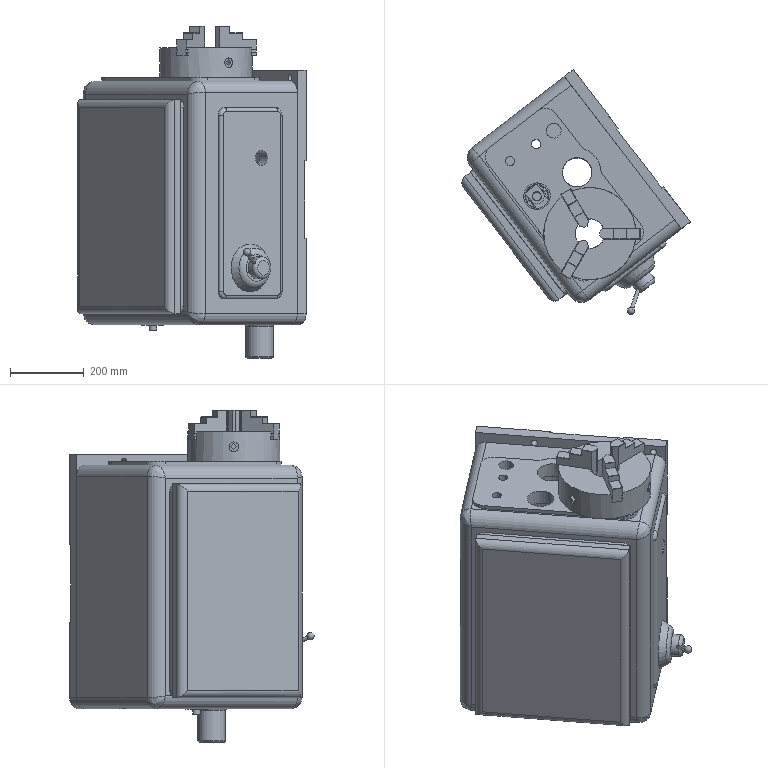Assembly | NX | mm | 12 component files | 21 solids | 565 faces | box 618.65 x 662.65 x 899.5 mm | volume 47575714 mm3 | plane 330 | cylinder 177 | torus 22 | spline 13 | cone 12 | sphere 11 | commonest cylinder face diameters 2 x32 25 x13 40 x13 70 x13 20 x13 80 x10 22 x9 60 x7
Bill of materials:
unnamed part 1 | 1 |  | Short, thick cylindrical disc with a central through-bore. The top face is split by three radial slots about 120 degrees apart, and small holes enter the outer cylindrical face.
unnamed part 2 | 1 |  | Rectangular box-shaped body with rounded edges. One face has five round through-holes of different sizes, the side faces have raised rectangular pads with small holes, a short cylindrical boss sticks out of the bottom, and flat plates are attached along one side.
unnamed part 3 | 1 |  | Bracket or lever with a cylindrical hub. The hub has a round bore with small notches around it. Two parallel flat plates stick out from the hub to form a fork-like gap, and a sloped triangular gusset supports them.
unnamed part 4 | 1 |  | Long, slender, straight cylindrical rod or pin with a short reduced-diameter step at one end.
unnamed part 5 | 1 |  | Thin rectangular plate with rounded edges. It has a narrow step or lip along one long edge and a narrow straight groove or strip parallel to one edge on one face.
unnamed part 6 | 2 |  | Annular part with a stepped outer diameter: a wider upper ring above a narrower lower ring. The top face has a concentric inner ring and an outer ring with an annular channel between them, and one small round element sits in the channel.
unnamed part 7 | 1 |  | Bracket with a vertical cylindrical hub. The hub has a bore with small notches around it, two parallel flat plates stick out sideways from the hub, a sloped triangular gusset sits above the upper plate, and a straight rib runs along the hub.
unnamed part 8 | 1 |  | Cone- or dish-shaped round base with a stepped cylindrical boss. A thin rod sticks out at an angle and ends in a small sphere. The surfaces are faceted.
unnamed part 9 | 3 |  | Solid block with a three-step staircase profile of increasing height. One end is chamfered or pointed in plan view, and a shallow groove or rebate runs along the lower part of the side faces.
Mates:
1. touch align | CA6140-zhou12-bocha1 1 face | CA6140-zhou12-huajianzhou 1
2. touch align | CA6140-zhou12-bocha1 1 face | CA6140-zhou12-huajianzhou 1
3. touch align | CA6140-zhou12-huajianzhou 1 | CA6140-zhou12-bocha2 1 face
4. touch align | CA6140-zhou12-bocha2 1 face | CA6140-zhou12-huajianzhou 1
5. touch align | assembly face | jaw 3 face
6. touch align | assembly face | jaw 3 face
7. touch align | jaw 3 face | assembly face
8. touch align | jaw 2 face | assembly face
9. touch align | jaw 2 face | assembly face
10. touch align | jaw 2 face | assembly face
11. touch align | assembly face | jaw 1 face
12. touch align | assembly face | jaw 1 face
13. touch align | assembly face | jaw 1 face
14. concentric | CA6140-zhou12-zhuangpei 1 edge | C6140-ZHOU4-zhoucheng2 1 edge